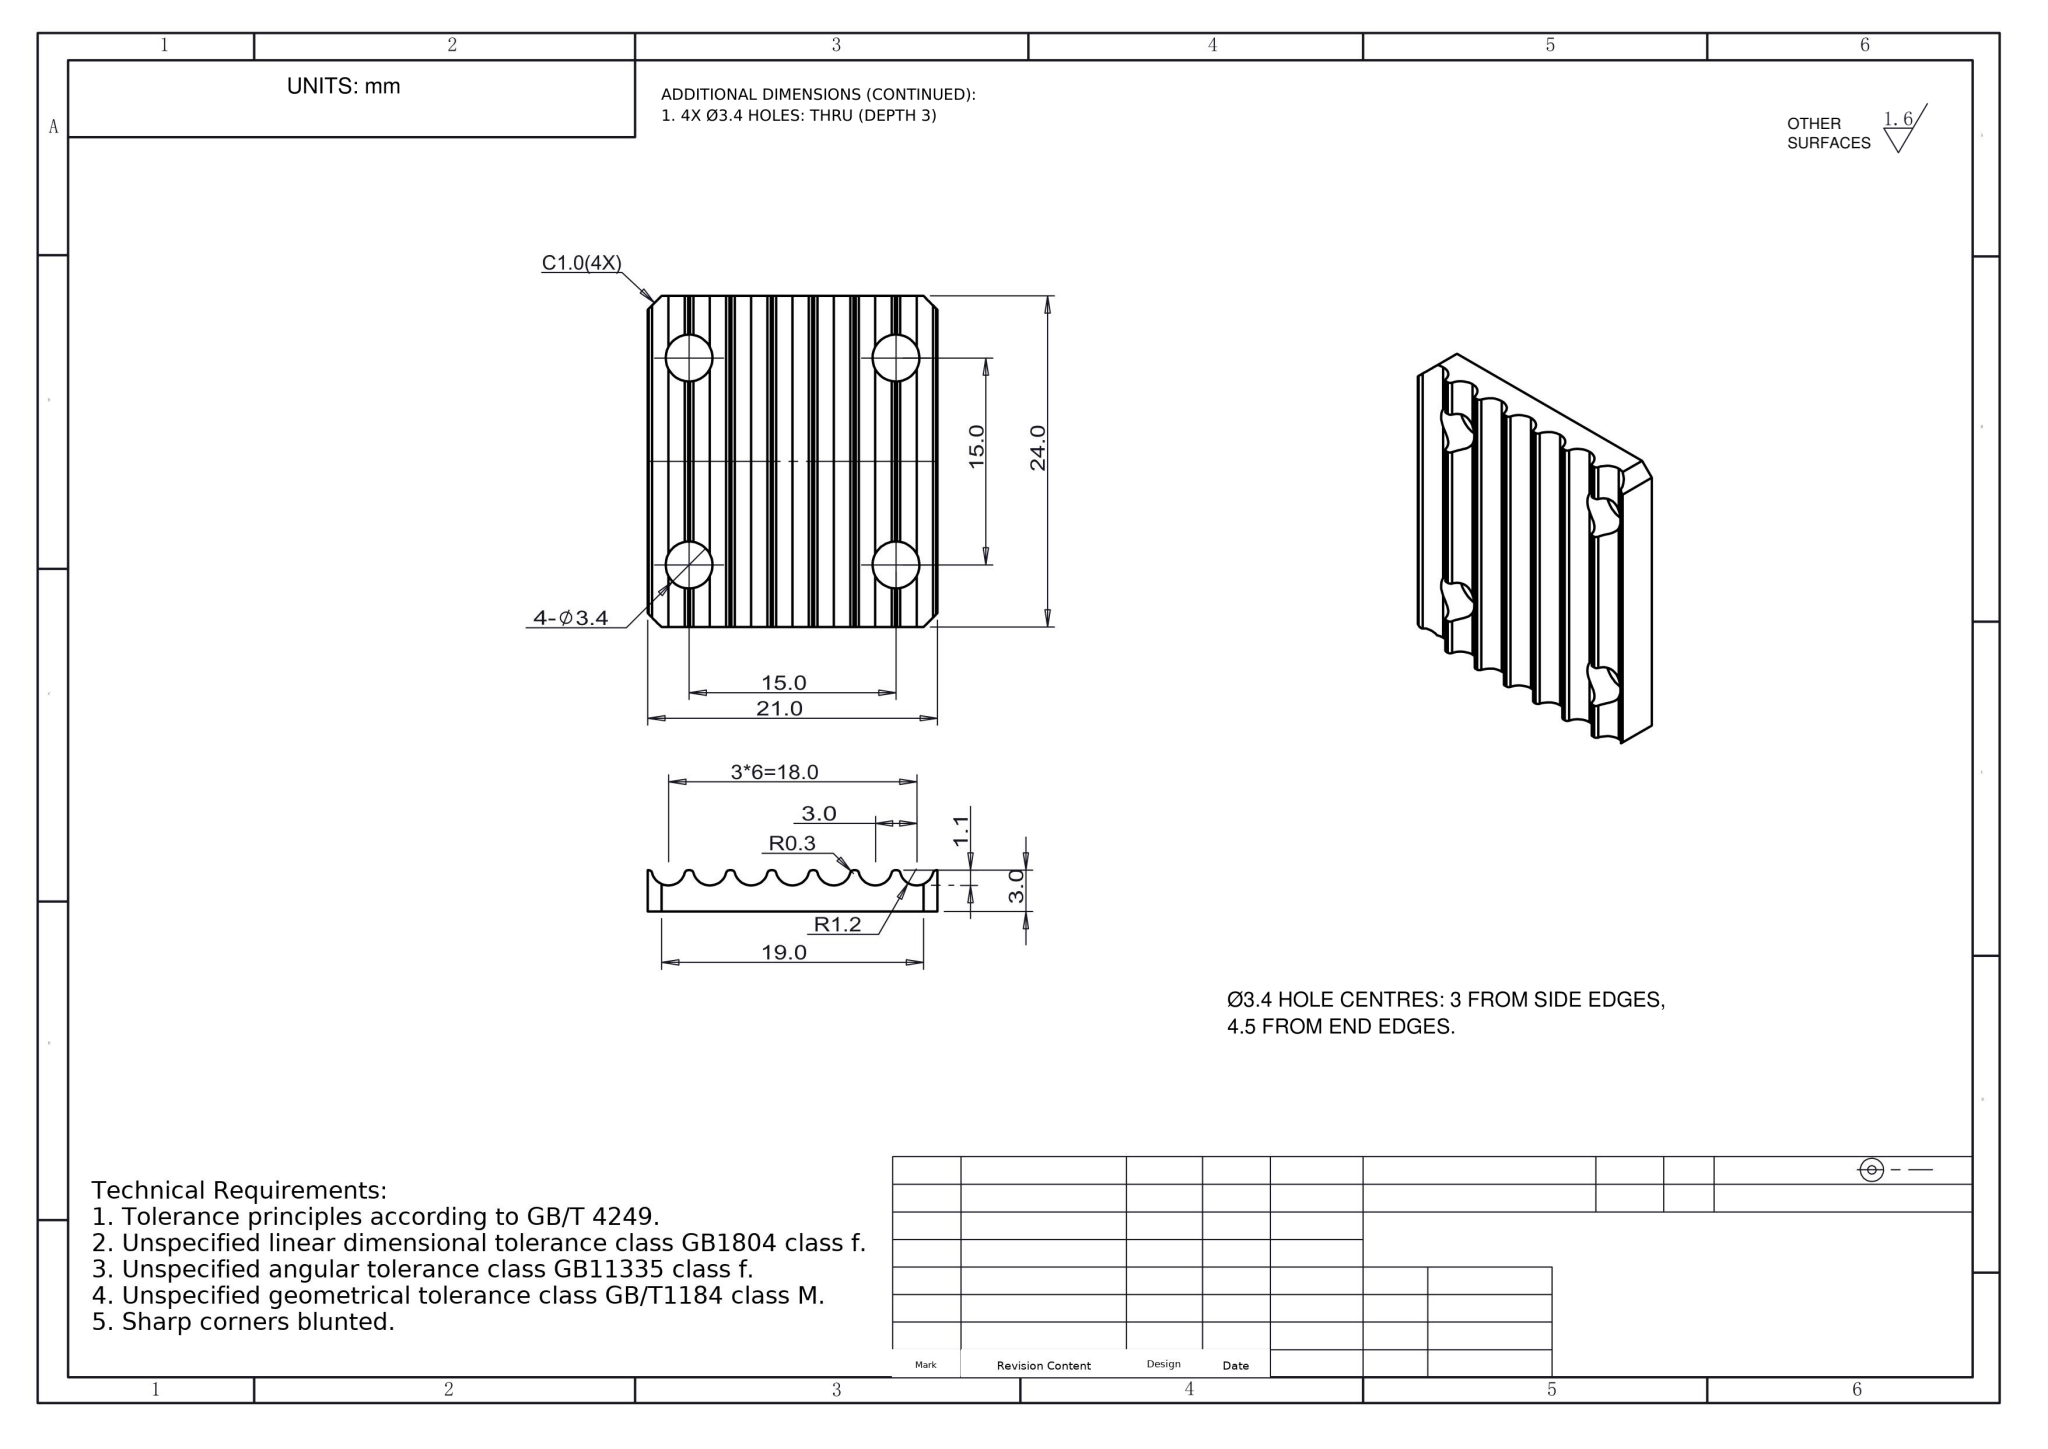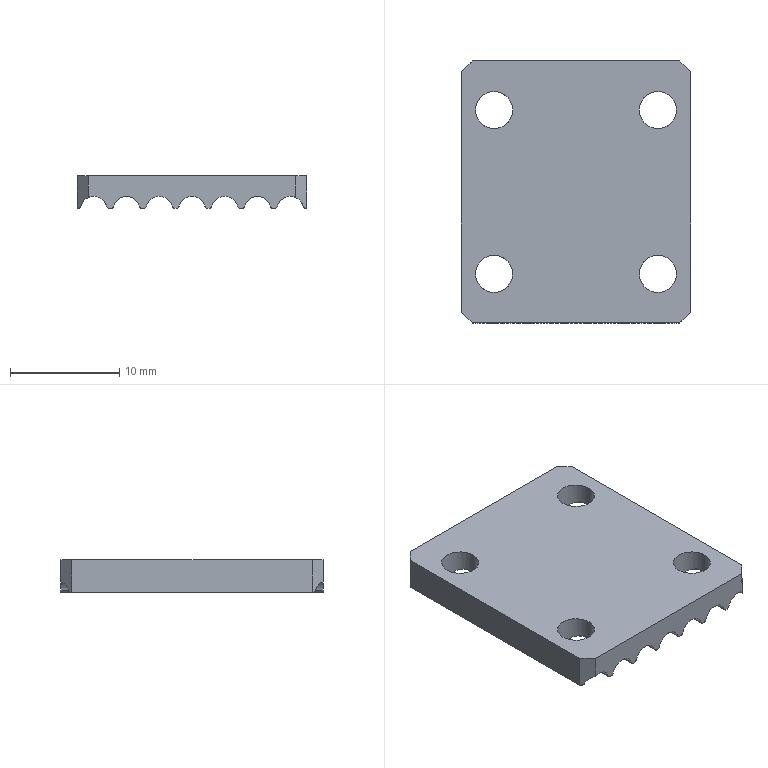Part | NX | mm | 1 solid | 103 faces | box 21 x 24 x 3 mm | volume 1072 mm3 | cylinder 82 | plane 21 | commonest cylinder face diameters 2.4 x52 0.5 x22 3.4 x8